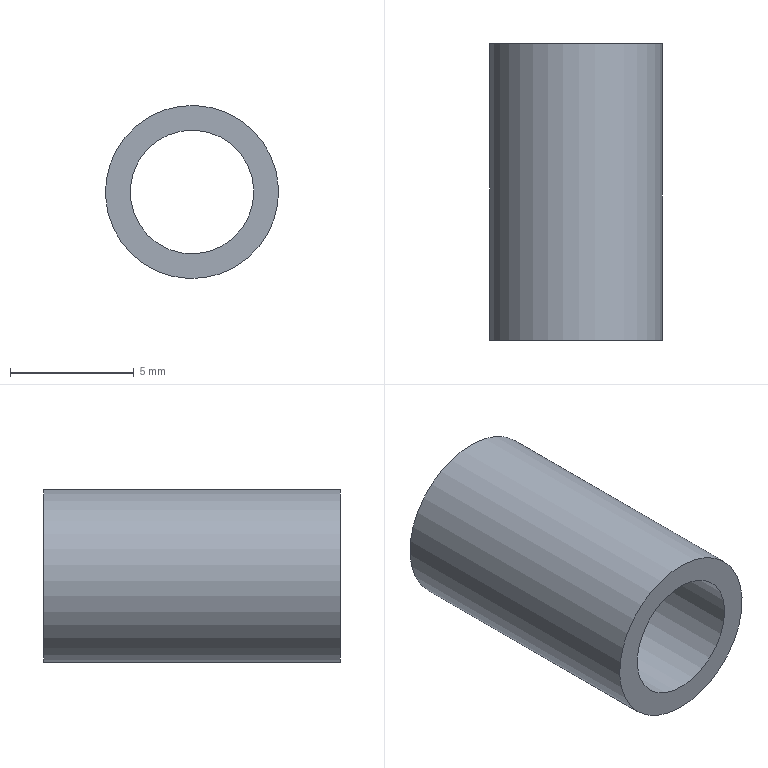Component | NX | TOP_BEARING_SHELL | 1 solid | 4 faces | volume 226 mm3 | cylinder 2 | plane 2 | commonest cylinder face diameters 7 x1 5 x1